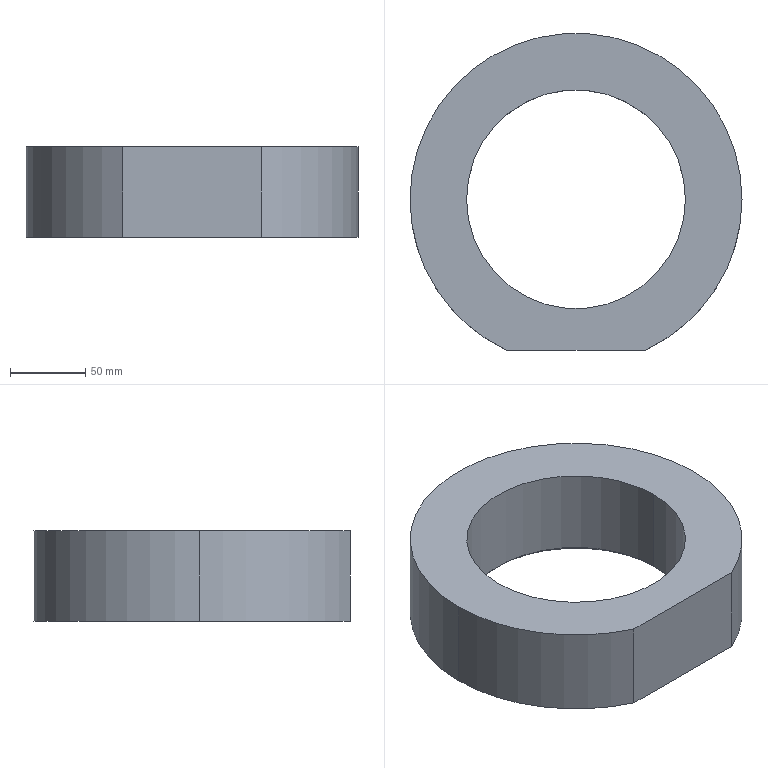Component | SolidWorks | JF21-80.1-1-3(_)-1-SOLID21-1 | 1 solid | 34 faces | box 220 x 210 x 60 mm | volume 1236758 mm3 | cylinder 17 | cone 14 | plane 3 | commonest cylinder face diameters 10.2 x12 220 x3 145 x2
STEP:
#1=CARTESIAN_POINT('',(2.854,-15.598,8.937));
#2=VERTEX_POINT('',#1);
#3=CARTESIAN_POINT('',(-2.854,-15.598,8.937));
#4=VERTEX_POINT('',#3);
#5=CARTESIAN_POINT('',(0.,-15.598,8.937));
#6=DIRECTION('',(0.,0.,-1.));
#7=DIRECTION('',(1.,0.,0.));
#8=AXIS2_PLACEMENT_3D('',#5,#6,#7);
#9=CIRCLE('',#8,2.854);
#10=EDGE_CURVE('',#2,#4,#9,.T.);
#11=ORIENTED_EDGE('',*,*,#10,.F.);
#12=CARTESIAN_POINT('',(2.933,-15.598,8.858));
#13=VERTEX_POINT('',#12);
#14=CARTESIAN_POINT('',(2.933,-15.598,8.858));
#15=DIRECTION('',(-0.7071,-0.,0.7071));
#16=VECTOR('',#15,39.37);
#17=LINE('',#14,#16);
#18=EDGE_CURVE('',#13,#2,#17,.T.);
#19=ORIENTED_EDGE('',*,*,#18,.F.);
#20=CARTESIAN_POINT('',(-2.933,-15.598,8.858));
#21=VERTEX_POINT('',#20);
#22=CARTESIAN_POINT('',(0.,-15.598,8.858));
#23=DIRECTION('',(0.,0.,1.));
#24=DIRECTION('',(1.,0.,0.));
#25=AXIS2_PLACEMENT_3D('',#22,#23,#24);
#26=CIRCLE('',#25,2.933);
#27=EDGE_CURVE('',#21,#13,#26,.T.);
#28=ORIENTED_EDGE('',*,*,#27,.F.);
#29=CARTESIAN_POINT('',(-2.933,-15.598,8.858));
#30=DIRECTION('',(0.7071,0.,0.7071));
#31=VECTOR('',#30,39.37);
#32=LINE('',#29,#31);
#33=EDGE_CURVE('',#21,#4,#32,.T.);
#34=ORIENTED_EDGE('',*,*,#33,.T.);
#35=EDGE_LOOP('',(#11,#19,#28,#34));
#36=FACE_OUTER_BOUND('',#35,.T.);
#37=CARTESIAN_POINT('',(0.,-15.598,8.858));
#38=DIRECTION('',(0.,0.,-1.));
#39=DIRECTION('',(1.,0.,0.));
#40=AXIS2_PLACEMENT_3D('',#37,#38,#39);
#41=CONICAL_SURFACE('',#40,2.933,0.7854);
#42=ADVANCED_FACE('',(#36),#41,.F.);
#43=CARTESIAN_POINT('',(3.269,-13.826,10.049));
#44=VERTEX_POINT('',#43);
#45=CARTESIAN_POINT('',(2.868,-13.826,10.049));
#46=VERTEX_POINT('',#45);
#47=CARTESIAN_POINT('',(3.069,-13.826,10.049));
#48=DIRECTION('',(0.,0.,-1.));
#49=DIRECTION('',(-1.,0.,0.));
#50=AXIS2_PLACEMENT_3D('',#47,#48,#49);
#51=CIRCLE('',#50,0.2008);
#52=EDGE_CURVE('',#44,#46,#51,.T.);
#53=ORIENTED_EDGE('',*,*,#52,.F.);
#54=CARTESIAN_POINT('',(3.269,-13.826,8.858));
#55=VERTEX_POINT('',#54);
#56=CARTESIAN_POINT('',(3.269,-13.826,8.858));
#57=DIRECTION('',(0.,0.,1.));
#58=VECTOR('',#57,39.37);
#59=LINE('',#56,#58);
#60=EDGE_CURVE('',#55,#44,#59,.T.);
#61=ORIENTED_EDGE('',*,*,#60,.F.);
#62=CARTESIAN_POINT('',(2.868,-13.826,8.858));
#63=VERTEX_POINT('',#62);
#64=CARTESIAN_POINT('',(3.069,-13.826,8.858));
#65=DIRECTION('',(0.,0.,-1.));
#66=DIRECTION('',(-1.,0.,0.));
#67=AXIS2_PLACEMENT_3D('',#64,#65,#66);
#68=CIRCLE('',#67,0.2008);
#69=EDGE_CURVE('',#55,#63,#68,.T.);
#70=ORIENTED_EDGE('',*,*,#69,.T.);
#71=CARTESIAN_POINT('',(2.868,-13.826,8.858));
#72=DIRECTION('',(0.,0.,1.));
#73=VECTOR('',#72,39.37);
#74=LINE('',#71,#73);
#75=EDGE_CURVE('',#63,#46,#74,.T.);
#76=ORIENTED_EDGE('',*,*,#75,.T.);
#77=EDGE_LOOP('',(#53,#61,#70,#76));
#78=FACE_OUTER_BOUND('',#77,.T.);
#79=CARTESIAN_POINT('',(3.069,-13.826,8.858));
#80=DIRECTION('',(0.,0.,-1.));
#81=DIRECTION('',(1.,0.,0.));
#82=AXIS2_PLACEMENT_3D('',#79,#80,#81);
#83=CYLINDRICAL_SURFACE('',#82,0.2008);
#84=ADVANCED_FACE('',(#78),#83,.F.);
#85=CARTESIAN_POINT('',(3.069,-13.826,10.17));
#86=VERTEX_POINT('',#85);
#87=CARTESIAN_POINT('',(2.868,-13.826,10.049));
#88=DIRECTION('',(0.8572,0.,0.515));
#89=VECTOR('',#88,39.37);
#90=LINE('',#87,#89);
#91=EDGE_CURVE('',#46,#86,#90,.T.);
#92=ORIENTED_EDGE('',*,*,#91,.T.);
#93=CARTESIAN_POINT('',(3.269,-13.826,10.049));
#94=DIRECTION('',(-0.8572,-0.,0.515));
#95=VECTOR('',#94,39.37);
#96=LINE('',#93,#95);
#97=EDGE_CURVE('',#44,#86,#96,.T.);
#98=ORIENTED_EDGE('',*,*,#97,.F.);
#99=ORIENTED_EDGE('',*,*,#52,.T.);
#100=EDGE_LOOP('',(#92,#98,#99));
#101=FACE_OUTER_BOUND('',#100,.T.);
#102=CARTESIAN_POINT('',(3.069,-13.826,10.049));
#103=DIRECTION('',(0.,0.,-1.));
#104=DIRECTION('',(1.,0.,0.));
#105=AXIS2_PLACEMENT_3D('',#102,#103,#104);
#106=CONICAL_SURFACE('',#105,0.2008,1.03);
#107=ADVANCED_FACE('',(#101),#106,.F.);
#108=CARTESIAN_POINT('',(3.269,-17.37,10.049));
#109=VERTEX_POINT('',#108);
#110=CARTESIAN_POINT('',(2.868,-17.37,10.049));
#111=VERTEX_POINT('',#110);
#112=CARTESIAN_POINT('',(3.069,-17.37,10.049));
#113=DIRECTION('',(0.,0.,-1.));
#114=DIRECTION('',(-1.,0.,0.));
#115=AXIS2_PLACEMENT_3D('',#112,#113,#114);
#116=CIRCLE('',#115,0.2008);
#117=EDGE_CURVE('',#109,#111,#116,.T.);
#118=ORIENTED_EDGE('',*,*,#117,.F.);
#119=CARTESIAN_POINT('',(3.269,-17.37,8.858));
#120=VERTEX_POINT('',#119);
#121=CARTESIAN_POINT('',(3.269,-17.37,8.858));
#122=DIRECTION('',(0.,0.,1.));
#123=VECTOR('',#122,39.37);
#124=LINE('',#121,#123);
#125=EDGE_CURVE('',#120,#109,#124,.T.);
#126=ORIENTED_EDGE('',*,*,#125,.F.);
#127=CARTESIAN_POINT('',(2.868,-17.37,8.858));
#128=VERTEX_POINT('',#127);
#129=CARTESIAN_POINT('',(3.069,-17.37,8.858));
#130=DIRECTION('',(0.,0.,-1.));
#131=DIRECTION('',(-1.,0.,0.));
#132=AXIS2_PLACEMENT_3D('',#129,#130,#131);
#133=CIRCLE('',#132,0.2008);
#134=EDGE_CURVE('',#120,#128,#133,.T.);
#135=ORIENTED_EDGE('',*,*,#134,.T.);
#136=CARTESIAN_POINT('',(2.868,-17.37,8.858));
#137=DIRECTION('',(0.,0.,1.));
#138=VECTOR('',#137,39.37);
#139=LINE('',#136,#138);
#140=EDGE_CURVE('',#128,#111,#139,.T.);
#141=ORIENTED_EDGE('',*,*,#140,.T.);
#142=EDGE_LOOP('',(#118,#126,#135,#141));
#143=FACE_OUTER_BOUND('',#142,.T.);
#144=CARTESIAN_POINT('',(3.069,-17.37,8.858));
#145=DIRECTION('',(0.,0.,-1.));
#146=DIRECTION('',(1.,0.,0.));
#147=AXIS2_PLACEMENT_3D('',#144,#145,#146);
#148=CYLINDRICAL_SURFACE('',#147,0.2008);
#149=ADVANCED_FACE('',(#143),#148,.F.);
#150=CARTESIAN_POINT('',(3.069,-17.37,10.17));
#151=VERTEX_POINT('',#150);
#152=CARTESIAN_POINT('',(2.868,-17.37,10.049));
#153=DIRECTION('',(0.8572,0.,0.515));
#154=VECTOR('',#153,39.37);
#155=LINE('',#152,#154);
#156=EDGE_CURVE('',#111,#151,#155,.T.);
#157=ORIENTED_EDGE('',*,*,#156,.T.);
#158=CARTESIAN_POINT('',(3.269,-17.37,10.049));
#159=DIRECTION('',(-0.8572,-0.,0.515));
#160=VECTOR('',#159,39.37);
#161=LINE('',#158,#160);
#162=EDGE_CURVE('',#109,#151,#161,.T.);
#163=ORIENTED_EDGE('',*,*,#162,.F.);
#164=ORIENTED_EDGE('',*,*,#117,.T.);
#165=EDGE_LOOP('',(#157,#163,#164));
#166=FACE_OUTER_BOUND('',#165,.T.);
#167=CARTESIAN_POINT('',(3.069,-17.37,10.049));
#168=DIRECTION('',(0.,0.,-1.));
#169=DIRECTION('',(1.,0.,0.));
#170=AXIS2_PLACEMENT_3D('',#167,#168,#169);
#171=CONICAL_SURFACE('',#170,0.2008,1.03);
#172=ADVANCED_FACE('',(#166),#171,.F.);
#173=CARTESIAN_POINT('',(0.2008,-19.141,10.049));
#174=VERTEX_POINT('',#173);
#175=CARTESIAN_POINT('',(-0.2008,-19.141,10.049));
#176=VERTEX_POINT('',#175);
#177=CARTESIAN_POINT('',(0.,-19.141,10.049));
#178=DIRECTION('',(0.,0.,-1.));
#179=DIRECTION('',(-1.,0.,0.));
#180=AXIS2_PLACEMENT_3D('',#177,#178,#179);
#181=CIRCLE('',#180,0.2008);
#182=EDGE_CURVE('',#174,#176,#181,.T.);
#183=ORIENTED_EDGE('',*,*,#182,.F.);
#184=CARTESIAN_POINT('',(0.2008,-19.141,8.858));
#185=VERTEX_POINT('',#184);
#186=CARTESIAN_POINT('',(0.2008,-19.141,8.858));
#187=DIRECTION('',(0.,0.,1.));
#188=VECTOR('',#187,39.37);
#189=LINE('',#186,#188);
#190=EDGE_CURVE('',#185,#174,#189,.T.);
#191=ORIENTED_EDGE('',*,*,#190,.F.);
#192=CARTESIAN_POINT('',(-0.2008,-19.141,8.858));
#193=VERTEX_POINT('',#192);
#194=CARTESIAN_POINT('',(0.,-19.141,8.858));
#195=DIRECTION('',(0.,0.,-1.));
#196=DIRECTION('',(-1.,0.,0.));
#197=AXIS2_PLACEMENT_3D('',#194,#195,#196);
#198=CIRCLE('',#197,0.2008);
#199=EDGE_CURVE('',#185,#193,#198,.T.);
#200=ORIENTED_EDGE('',*,*,#199,.T.);
#201=CARTESIAN_POINT('',(-0.2008,-19.141,8.858));
#202=DIRECTION('',(0.,0.,1.));
#203=VECTOR('',#202,39.37);
#204=LINE('',#201,#203);
#205=EDGE_CURVE('',#193,#176,#204,.T.);
#206=ORIENTED_EDGE('',*,*,#205,.T.);
#207=EDGE_LOOP('',(#183,#191,#200,#206));
#208=FACE_OUTER_BOUND('',#207,.T.);
#209=CARTESIAN_POINT('',(0.,-19.141,8.858));
#210=DIRECTION('',(0.,0.,-1.));
#211=DIRECTION('',(1.,0.,0.));
#212=AXIS2_PLACEMENT_3D('',#209,#210,#211);
#213=CYLINDRICAL_SURFACE('',#212,0.2008);
#214=ADVANCED_FACE('',(#208),#213,.F.);
#215=CARTESIAN_POINT('',(0.,-19.141,10.17));
#216=VERTEX_POINT('',#215);
#217=CARTESIAN_POINT('',(-0.2008,-19.141,10.049));
#218=DIRECTION('',(0.8572,0.,0.515));
#219=VECTOR('',#218,39.37);
#220=LINE('',#217,#219);
#221=EDGE_CURVE('',#176,#216,#220,.T.);
#222=ORIENTED_EDGE('',*,*,#221,.T.);
#223=CARTESIAN_POINT('',(0.2008,-19.141,10.049));
#224=DIRECTION('',(-0.8572,-0.,0.515));
#225=VECTOR('',#224,39.37);
#226=LINE('',#223,#225);
#227=EDGE_CURVE('',#174,#216,#226,.T.);
#228=ORIENTED_EDGE('',*,*,#227,.F.);
#229=ORIENTED_EDGE('',*,*,#182,.T.);
#230=EDGE_LOOP('',(#222,#228,#229));
#231=FACE_OUTER_BOUND('',#230,.T.);
#232=CARTESIAN_POINT('',(0.,-19.141,10.049));
#233=DIRECTION('',(0.,0.,-1.));
#234=DIRECTION('',(1.,0.,0.));
#235=AXIS2_PLACEMENT_3D('',#232,#233,#234);
#236=CONICAL_SURFACE('',#235,0.2008,1.03);
#237=ADVANCED_FACE('',(#231),#236,.F.);
#238=CARTESIAN_POINT('',(-2.868,-17.37,10.049));
#239=VERTEX_POINT('',#238);
#240=CARTESIAN_POINT('',(-3.269,-17.37,10.049));
#241=VERTEX_POINT('',#240);
#242=CARTESIAN_POINT('',(-3.069,-17.37,10.049));
#243=DIRECTION('',(0.,0.,-1.));
#244=DIRECTION('',(-1.,0.,0.));
#245=AXIS2_PLACEMENT_3D('',#242,#243,#244);
#246=CIRCLE('',#245,0.2008);
#247=EDGE_CURVE('',#239,#241,#246,.T.);
#248=ORIENTED_EDGE('',*,*,#247,.F.);
#249=CARTESIAN_POINT('',(-2.868,-17.37,8.858));
#250=VERTEX_POINT('',#249);
#251=CARTESIAN_POINT('',(-2.868,-17.37,8.858));
#252=DIRECTION('',(0.,0.,1.));
#253=VECTOR('',#252,39.37);
#254=LINE('',#251,#253);
#255=EDGE_CURVE('',#250,#239,#254,.T.);
#256=ORIENTED_EDGE('',*,*,#255,.F.);
#257=CARTESIAN_POINT('',(-3.269,-17.37,8.858));
#258=VERTEX_POINT('',#257);
#259=CARTESIAN_POINT('',(-3.069,-17.37,8.858));
#260=DIRECTION('',(0.,0.,-1.));
#261=DIRECTION('',(-1.,0.,0.));
#262=AXIS2_PLACEMENT_3D('',#259,#260,#261);
#263=CIRCLE('',#262,0.2008);
#264=EDGE_CURVE('',#250,#258,#263,.T.);
#265=ORIENTED_EDGE('',*,*,#264,.T.);
#266=CARTESIAN_POINT('',(-3.269,-17.37,8.858));
#267=DIRECTION('',(0.,0.,1.));
#268=VECTOR('',#267,39.37);
#269=LINE('',#266,#268);
#270=EDGE_CURVE('',#258,#241,#269,.T.);
#271=ORIENTED_EDGE('',*,*,#270,.T.);
#272=EDGE_LOOP('',(#248,#256,#265,#271));
#273=FACE_OUTER_BOUND('',#272,.T.);
#274=CARTESIAN_POINT('',(-3.069,-17.37,8.858));
#275=DIRECTION('',(0.,0.,-1.));
#276=DIRECTION('',(1.,0.,0.));
#277=AXIS2_PLACEMENT_3D('',#274,#275,#276);
#278=CYLINDRICAL_SURFACE('',#277,0.2008);
#279=ADVANCED_FACE('',(#273),#278,.F.);
#280=CARTESIAN_POINT('',(-3.069,-17.37,10.17));
#281=VERTEX_POINT('',#280);
#282=CARTESIAN_POINT('',(-3.269,-17.37,10.049));
#283=DIRECTION('',(0.8572,0.,0.515));
#284=VECTOR('',#283,39.37);
#285=LINE('',#282,#284);
#286=EDGE_CURVE('',#241,#281,#285,.T.);
#287=ORIENTED_EDGE('',*,*,#286,.T.);
#288=CARTESIAN_POINT('',(-2.868,-17.37,10.049));
#289=DIRECTION('',(-0.8572,-0.,0.515));
#290=VECTOR('',#289,39.37);
#291=LINE('',#288,#290);
#292=EDGE_CURVE('',#239,#281,#291,.T.);
#293=ORIENTED_EDGE('',*,*,#292,.F.);
#294=ORIENTED_EDGE('',*,*,#247,.T.);
#295=EDGE_LOOP('',(#287,#293,#294));
#296=FACE_OUTER_BOUND('',#295,.T.);
#297=CARTESIAN_POINT('',(-3.069,-17.37,10.049));
#298=DIRECTION('',(0.,0.,-1.));
#299=DIRECTION('',(1.,0.,0.));
#300=AXIS2_PLACEMENT_3D('',#297,#298,#299);
#301=CONICAL_SURFACE('',#300,0.2008,1.03);
#302=ADVANCED_FACE('',(#296),#301,.F.);
#303=CARTESIAN_POINT('',(-2.868,-13.826,10.049));
#304=VERTEX_POINT('',#303);
#305=CARTESIAN_POINT('',(-3.269,-13.826,10.049));
#306=VERTEX_POINT('',#305);
#307=CARTESIAN_POINT('',(-3.069,-13.826,10.049));
#308=DIRECTION('',(0.,0.,-1.));
#309=DIRECTION('',(-1.,0.,0.));
#310=AXIS2_PLACEMENT_3D('',#307,#308,#309);
#311=CIRCLE('',#310,0.2008);
#312=EDGE_CURVE('',#304,#306,#311,.T.);
#313=ORIENTED_EDGE('',*,*,#312,.F.);
#314=CARTESIAN_POINT('',(-2.868,-13.826,8.858));
#315=VERTEX_POINT('',#314);
#316=CARTESIAN_POINT('',(-2.868,-13.826,8.858));
#317=DIRECTION('',(0.,0.,1.));
#318=VECTOR('',#317,39.37);
#319=LINE('',#316,#318);
#320=EDGE_CURVE('',#315,#304,#319,.T.);
#321=ORIENTED_EDGE('',*,*,#320,.F.);
#322=CARTESIAN_POINT('',(-3.269,-13.826,8.858));
#323=VERTEX_POINT('',#322);
#324=CARTESIAN_POINT('',(-3.069,-13.826,8.858));
#325=DIRECTION('',(0.,0.,-1.));
#326=DIRECTION('',(-1.,0.,0.));
#327=AXIS2_PLACEMENT_3D('',#324,#325,#326);
#328=CIRCLE('',#327,0.2008);
#329=EDGE_CURVE('',#315,#323,#328,.T.);
#330=ORIENTED_EDGE('',*,*,#329,.T.);
#331=CARTESIAN_POINT('',(-3.269,-13.826,8.858));
#332=DIRECTION('',(0.,0.,1.));
#333=VECTOR('',#332,39.37);
#334=LINE('',#331,#333);
#335=EDGE_CURVE('',#323,#306,#334,.T.);
#336=ORIENTED_EDGE('',*,*,#335,.T.);
#337=EDGE_LOOP('',(#313,#321,#330,#336));
#338=FACE_OUTER_BOUND('',#337,.T.);
#339=CARTESIAN_POINT('',(-3.069,-13.826,8.858));
#340=DIRECTION('',(0.,0.,-1.));
#341=DIRECTION('',(1.,0.,0.));
#342=AXIS2_PLACEMENT_3D('',#339,#340,#341);
#343=CYLINDRICAL_SURFACE('',#342,0.2008);
#344=ADVANCED_FACE('',(#338),#343,.F.);
#345=CARTESIAN_POINT('',(-3.069,-13.826,10.17));
#346=VERTEX_POINT('',#345);
#347=CARTESIAN_POINT('',(-3.269,-13.826,10.049));
#348=DIRECTION('',(0.8572,0.,0.515));
#349=VECTOR('',#348,39.37);
#350=LINE('',#347,#349);
#351=EDGE_CURVE('',#306,#346,#350,.T.);
#352=ORIENTED_EDGE('',*,*,#351,.T.);
#353=CARTESIAN_POINT('',(-2.868,-13.826,10.049));
#354=DIRECTION('',(-0.8572,-0.,0.515));
#355=VECTOR('',#354,39.37);
#356=LINE('',#353,#355);
#357=EDGE_CURVE('',#304,#346,#356,.T.);
#358=ORIENTED_EDGE('',*,*,#357,.F.);
#359=ORIENTED_EDGE('',*,*,#312,.T.);
#360=EDGE_LOOP('',(#352,#358,#359));
#361=FACE_OUTER_BOUND('',#360,.T.);
#362=CARTESIAN_POINT('',(-3.069,-13.826,10.049));
#363=DIRECTION('',(0.,0.,-1.));
#364=DIRECTION('',(1.,0.,0.));
#365=AXIS2_PLACEMENT_3D('',#362,#363,#364);
#366=CONICAL_SURFACE('',#365,0.2008,1.03);
#367=ADVANCED_FACE('',(#361),#366,.F.);
#368=CARTESIAN_POINT('',(0.2008,-12.055,10.049));
#369=VERTEX_POINT('',#368);
#370=CARTESIAN_POINT('',(-0.2008,-12.055,10.049));
#371=VERTEX_POINT('',#370);
#372=CARTESIAN_POINT('',(0.,-12.055,10.049));
#373=DIRECTION('',(0.,0.,-1.));
#374=DIRECTION('',(-1.,0.,0.));
#375=AXIS2_PLACEMENT_3D('',#372,#373,#374);
#376=CIRCLE('',#375,0.2008);
#377=EDGE_CURVE('',#369,#371,#376,.T.);
#378=ORIENTED_EDGE('',*,*,#377,.F.);
#379=CARTESIAN_POINT('',(0.2008,-12.055,8.858));
#380=VERTEX_POINT('',#379);
#381=CARTESIAN_POINT('',(0.2008,-12.055,8.858));
#382=DIRECTION('',(0.,0.,1.));
#383=VECTOR('',#382,39.37);
#384=LINE('',#381,#383);
#385=EDGE_CURVE('',#380,#369,#384,.T.);
#386=ORIENTED_EDGE('',*,*,#385,.F.);
#387=CARTESIAN_POINT('',(-0.2008,-12.055,8.858));
#388=VERTEX_POINT('',#387);
#389=CARTESIAN_POINT('',(0.,-12.055,8.858));
#390=DIRECTION('',(0.,0.,-1.));
#391=DIRECTION('',(-1.,0.,0.));
#392=AXIS2_PLACEMENT_3D('',#389,#390,#391);
#393=CIRCLE('',#392,0.2008);
#394=EDGE_CURVE('',#380,#388,#393,.T.);
#395=ORIENTED_EDGE('',*,*,#394,.T.);
#396=CARTESIAN_POINT('',(-0.2008,-12.055,8.858));
#397=DIRECTION('',(0.,0.,1.));
#398=VECTOR('',#397,39.37);
#399=LINE('',#396,#398);
#400=EDGE_CURVE('',#388,#371,#399,.T.);
#401=ORIENTED_EDGE('',*,*,#400,.T.);
#402=EDGE_LOOP('',(#378,#386,#395,#401));
#403=FACE_OUTER_BOUND('',#402,.T.);
#404=CARTESIAN_POINT('',(0.,-12.055,8.858));
#405=DIRECTION('',(0.,0.,-1.));
#406=DIRECTION('',(1.,0.,0.));
#407=AXIS2_PLACEMENT_3D('',#404,#405,#406);
#408=CYLINDRICAL_SURFACE('',#407,0.2008);
#409=ADVANCED_FACE('',(#403),#408,.F.);
#410=CARTESIAN_POINT('',(-0.,-12.055,10.17));
#411=VERTEX_POINT('',#410);
#412=CARTESIAN_POINT('',(-0.2008,-12.055,10.049));
#413=DIRECTION('',(0.8572,0.,0.515));
#414=VECTOR('',#413,39.37);
#415=LINE('',#412,#414);
#416=EDGE_CURVE('',#371,#411,#415,.T.);
#417=ORIENTED_EDGE('',*,*,#416,.T.);
#418=CARTESIAN_POINT('',(0.2008,-12.055,10.049));
#419=DIRECTION('',(-0.8572,-0.,0.515));
#420=VECTOR('',#419,39.37);
#421=LINE('',#418,#420);
#422=EDGE_CURVE('',#369,#411,#421,.T.);
#423=ORIENTED_EDGE('',*,*,#422,.F.);
#424=ORIENTED_EDGE('',*,*,#377,.T.);
#425=EDGE_LOOP('',(#417,#423,#424));
#426=FACE_OUTER_BOUND('',#425,.T.);
#427=CARTESIAN_POINT('',(0.,-12.055,10.049));
#428=DIRECTION('',(0.,0.,-1.));
#429=DIRECTION('',(1.,0.,0.));
#430=AXIS2_PLACEMENT_3D('',#427,#428,#429);
#431=CONICAL_SURFACE('',#430,0.2008,1.03);
#432=ADVANCED_FACE('',(#426),#431,.F.);
#433=ORIENTED_EDGE('',*,*,#10,.T.);
#434=CARTESIAN_POINT('',(-2.854,-15.598,11.22));
#435=VERTEX_POINT('',#434);
#436=CARTESIAN_POINT('',(-2.854,-15.598,8.858));
#437=DIRECTION('',(0.,0.,1.));
#438=VECTOR('',#437,39.37);
#439=LINE('',#436,#438);
#440=EDGE_CURVE('',#4,#435,#439,.T.);
#441=ORIENTED_EDGE('',*,*,#440,.T.);
#442=CARTESIAN_POINT('',(2.854,-15.598,11.22));
#443=VERTEX_POINT('',#442);
#444=CARTESIAN_POINT('',(0.,-15.598,11.22));
#445=DIRECTION('',(0.,0.,1.));
#446=DIRECTION('',(1.,0.,0.));
#447=AXIS2_PLACEMENT_3D('',#444,#445,#446);
#448=CIRCLE('',#447,2.854);
#449=EDGE_CURVE('',#435,#443,#448,.T.);
#450=ORIENTED_EDGE('',*,*,#449,.T.);
#451=CARTESIAN_POINT('',(2.854,-15.598,8.858));
#452=DIRECTION('',(0.,0.,1.));
#453=VECTOR('',#452,39.37);
#454=LINE('',#451,#453);
#455=EDGE_CURVE('',#2,#443,#454,.T.);
#456=ORIENTED_EDGE('',*,*,#455,.F.);
#457=EDGE_LOOP('',(#433,#441,#450,#456));
#458=FACE_OUTER_BOUND('',#457,.T.);
#459=CARTESIAN_POINT('',(0.,-15.598,8.858));
#460=DIRECTION('',(0.,0.,1.));
#461=DIRECTION('',(-1.,0.,0.));
#462=AXIS2_PLACEMENT_3D('',#459,#460,#461);
#463=CYLINDRICAL_SURFACE('',#462,2.854);
#464=ADVANCED_FACE('',(#458),#463,.F.);
#465=CARTESIAN_POINT('',(4.331,-15.598,8.858));
#466=VERTEX_POINT('',#465);
#467=CARTESIAN_POINT('',(-4.331,-15.598,8.858));
#468=VERTEX_POINT('',#467);
#469=CARTESIAN_POINT('',(0.,-15.598,8.858));
#470=DIRECTION('',(0.,0.,1.));
#471=DIRECTION('',(1.,0.,0.));
#472=AXIS2_PLACEMENT_3D('',#469,#470,#471);
#473=CIRCLE('',#472,4.331);
#474=EDGE_CURVE('',#466,#468,#473,.T.);
#475=ORIENTED_EDGE('',*,*,#474,.T.);
#476=CARTESIAN_POINT('',(-4.331,-15.598,11.22));
#477=VERTEX_POINT('',#476);
#478=CARTESIAN_POINT('',(-4.331,-15.598,8.858));
#479=DIRECTION('',(0.,0.,1.));
#480=VECTOR('',#479,39.37);
#481=LINE('',#478,#480);
#482=EDGE_CURVE('',#468,#477,#481,.T.);
#483=ORIENTED_EDGE('',*,*,#482,.T.);
#484=CARTESIAN_POINT('',(4.331,-15.598,11.22));
#485=VERTEX_POINT('',#484);
#486=CARTESIAN_POINT('',(0.,-15.598,11.22));
#487=DIRECTION('',(0.,0.,1.));
#488=DIRECTION('',(1.,0.,0.));
#489=AXIS2_PLACEMENT_3D('',#486,#487,#488);
#490=CIRCLE('',#489,4.331);
#491=EDGE_CURVE('',#485,#477,#490,.T.);
#492=ORIENTED_EDGE('',*,*,#491,.F.);
#493=CARTESIAN_POINT('',(4.331,-15.598,8.858));
#494=DIRECTION('',(0.,0.,1.));
#495=VECTOR('',#494,39.37);
#496=LINE('',#493,#495);
#497=EDGE_CURVE('',#466,#485,#496,.T.);
#498=ORIENTED_EDGE('',*,*,#497,.F.);
#499=EDGE_LOOP('',(#475,#483,#492,#498));
#500=FACE_OUTER_BOUND('',#499,.T.);
#501=CARTESIAN_POINT('',(0.,-15.598,8.858));
#502=DIRECTION('',(0.,0.,1.));
#503=DIRECTION('',(-1.,0.,0.));
#504=AXIS2_PLACEMENT_3D('',#501,#502,#503);
#505=CYLINDRICAL_SURFACE('',#504,4.331);
#506=ADVANCED_FACE('',(#500),#505,.T.);
#507=CARTESIAN_POINT('',(1.804,-19.535,8.858));
#508=VERTEX_POINT('',#507);
#509=CARTESIAN_POINT('',(0.,-15.598,8.858));
#510=DIRECTION('',(0.,0.,1.));
#511=DIRECTION('',(1.,0.,0.));
#512=AXIS2_PLACEMENT_3D('',#509,#510,#511);
#513=CIRCLE('',#512,4.331);
#514=EDGE_CURVE('',#508,#466,#513,.T.);
#515=ORIENTED_EDGE('',*,*,#514,.T.);
#516=ORIENTED_EDGE('',*,*,#497,.T.);
#517=CARTESIAN_POINT('',(1.804,-19.535,11.22));
#518=VERTEX_POINT('',#517);
#519=CARTESIAN_POINT('',(0.,-15.598,11.22));
#520=DIRECTION('',(0.,0.,1.));
#521=DIRECTION('',(1.,0.,0.));
#522=AXIS2_PLACEMENT_3D('',#519,#520,#521);
#523=CIRCLE('',#522,4.331);
#524=EDGE_CURVE('',#518,#485,#523,.T.);
#525=ORIENTED_EDGE('',*,*,#524,.F.);
#526=CARTESIAN_POINT('',(1.804,-19.535,8.858));
#527=DIRECTION('',(0.,0.,1.));
#528=VECTOR('',#527,39.37);
#529=LINE('',#526,#528);
#530=EDGE_CURVE('',#508,#518,#529,.T.);
#531=ORIENTED_EDGE('',*,*,#530,.F.);
#532=EDGE_LOOP('',(#515,#516,#525,#531));
#533=FACE_OUTER_BOUND('',#532,.T.);
#534=CARTESIAN_POINT('',(0.,-15.598,8.858));
#535=DIRECTION('',(0.,0.,1.));
#536=DIRECTION('',(-1.,0.,0.));
#537=AXIS2_PLACEMENT_3D('',#534,#535,#536);
#538=CYLINDRICAL_SURFACE('',#537,4.331);
#539=ADVANCED_FACE('',(#533),#538,.T.);
#540=ORIENTED_EDGE('',*,*,#482,.F.);
#541=CARTESIAN_POINT('',(-1.804,-19.535,8.858));
#542=VERTEX_POINT('',#541);
#543=CARTESIAN_POINT('',(0.,-15.598,8.858));
#544=DIRECTION('',(0.,0.,1.));
#545=DIRECTION('',(1.,0.,0.));
#546=AXIS2_PLACEMENT_3D('',#543,#544,#545);
#547=CIRCLE('',#546,4.331);
#548=EDGE_CURVE('',#468,#542,#547,.T.);
#549=ORIENTED_EDGE('',*,*,#548,.T.);
#550=CARTESIAN_POINT('',(-1.804,-19.535,11.22));
#551=VERTEX_POINT('',#550);
#552=CARTESIAN_POINT('',(-1.804,-19.535,8.858));
#553=DIRECTION('',(0.,0.,1.));
#554=VECTOR('',#553,39.37);
#555=LINE('',#552,#554);
#556=EDGE_CURVE('',#542,#551,#555,.T.);
#557=ORIENTED_EDGE('',*,*,#556,.T.);
#558=CARTESIAN_POINT('',(0.,-15.598,11.22));
#559=DIRECTION('',(0.,0.,1.));
#560=DIRECTION('',(1.,0.,0.));
#561=AXIS2_PLACEMENT_3D('',#558,#559,#560);
#562=CIRCLE('',#561,4.331);
#563=EDGE_CURVE('',#477,#551,#562,.T.);
#564=ORIENTED_EDGE('',*,*,#563,.F.);
#565=EDGE_LOOP('',(#540,#549,#557,#564));
#566=FACE_OUTER_BOUND('',#565,.T.);
#567=CARTESIAN_POINT('',(0.,-15.598,8.858));
#568=DIRECTION('',(0.,0.,1.));
#569=DIRECTION('',(-1.,0.,0.));
#570=AXIS2_PLACEMENT_3D('',#567,#568,#569);
#571=CYLINDRICAL_SURFACE('',#570,4.331);
#572=ADVANCED_FACE('',(#566),#571,.T.);
#573=CARTESIAN_POINT('',(-1.804,-19.535,11.22));
#574=DIRECTION('',(1.,-0.,0.));
#575=VECTOR('',#574,39.37);
#576=LINE('',#573,#575);
#577=EDGE_CURVE('',#551,#518,#576,.T.);
#578=ORIENTED_EDGE('',*,*,#577,.F.);
#579=ORIENTED_EDGE('',*,*,#556,.F.);
#580=CARTESIAN_POINT('',(-1.804,-19.535,8.858));
#581=DIRECTION('',(1.,-0.,0.));
#582=VECTOR('',#581,39.37);
#583=LINE('',#580,#582);
#584=EDGE_CURVE('',#542,#508,#583,.T.);
#585=ORIENTED_EDGE('',*,*,#584,.T.);
#586=ORIENTED_EDGE('',*,*,#530,.T.);
#587=EDGE_LOOP('',(#578,#579,#585,#586));
#588=FACE_OUTER_BOUND('',#587,.T.);
#589=CARTESIAN_POINT('',(-1.804,-19.535,8.858));
#590=DIRECTION('',(-0.,-1.,0.));
#591=DIRECTION('',(-1.,0.,0.));
#592=AXIS2_PLACEMENT_3D('',#589,#590,#591);
#593=PLANE('',#592);
#594=ADVANCED_FACE('',(#588),#593,.T.);
#595=ORIENTED_EDGE('',*,*,#27,.T.);
#596=CARTESIAN_POINT('',(0.,-15.598,8.858));
#597=DIRECTION('',(0.,0.,1.));
#598=DIRECTION('',(1.,0.,0.));
#599=AXIS2_PLACEMENT_3D('',#596,#597,#598);
#600=CIRCLE('',#599,2.933);
#601=EDGE_CURVE('',#13,#21,#600,.T.);
#602=ORIENTED_EDGE('',*,*,#601,.T.);
#603=EDGE_LOOP('',(#595,#602));
#604=FACE_BOUND('',#603,.T.);
#605=CARTESIAN_POINT('',(3.069,-13.826,8.858));
#606=DIRECTION('',(0.,0.,-1.));
#607=DIRECTION('',(-1.,0.,0.));
#608=AXIS2_PLACEMENT_3D('',#605,#606,#607);
#609=CIRCLE('',#608,0.2008);
#610=EDGE_CURVE('',#63,#55,#609,.T.);
#611=ORIENTED_EDGE('',*,*,#610,.F.);
#612=ORIENTED_EDGE('',*,*,#69,.F.);
#613=EDGE_LOOP('',(#611,#612));
#614=FACE_BOUND('',#613,.T.);
#615=CARTESIAN_POINT('',(3.069,-17.37,8.858));
#616=DIRECTION('',(0.,0.,-1.));
#617=DIRECTION('',(-1.,0.,0.));
#618=AXIS2_PLACEMENT_3D('',#615,#616,#617);
#619=CIRCLE('',#618,0.2008);
#620=EDGE_CURVE('',#128,#120,#619,.T.);
#621=ORIENTED_EDGE('',*,*,#620,.F.);
#622=ORIENTED_EDGE('',*,*,#134,.F.);
#623=EDGE_LOOP('',(#621,#622));
#624=FACE_BOUND('',#623,.T.);
#625=CARTESIAN_POINT('',(0.,-19.141,8.858));
#626=DIRECTION('',(0.,0.,-1.));
#627=DIRECTION('',(-1.,0.,0.));
#628=AXIS2_PLACEMENT_3D('',#625,#626,#627);
#629=CIRCLE('',#628,0.2008);
#630=EDGE_CURVE('',#193,#185,#629,.T.);
#631=ORIENTED_EDGE('',*,*,#630,.F.);
#632=ORIENTED_EDGE('',*,*,#199,.F.);
#633=EDGE_LOOP('',(#631,#632));
#634=FACE_BOUND('',#633,.T.);
#635=CARTESIAN_POINT('',(-3.069,-17.37,8.858));
#636=DIRECTION('',(0.,0.,-1.));
#637=DIRECTION('',(-1.,0.,0.));
#638=AXIS2_PLACEMENT_3D('',#635,#636,#637);
#639=CIRCLE('',#638,0.2008);
#640=EDGE_CURVE('',#258,#250,#639,.T.);
#641=ORIENTED_EDGE('',*,*,#640,.F.);
#642=ORIENTED_EDGE('',*,*,#264,.F.);
#643=EDGE_LOOP('',(#641,#642));
#644=FACE_BOUND('',#643,.T.);
#645=CARTESIAN_POINT('',(-3.069,-13.826,8.858));
#646=DIRECTION('',(0.,0.,-1.));
#647=DIRECTION('',(-1.,0.,0.));
#648=AXIS2_PLACEMENT_3D('',#645,#646,#647);
#649=CIRCLE('',#648,0.2008);
#650=EDGE_CURVE('',#323,#315,#649,.T.);
#651=ORIENTED_EDGE('',*,*,#650,.F.);
#652=ORIENTED_EDGE('',*,*,#329,.F.);
#653=EDGE_LOOP('',(#651,#652));
#654=FACE_BOUND('',#653,.T.);
#655=CARTESIAN_POINT('',(0.,-12.055,8.858));
#656=DIRECTION('',(0.,0.,-1.));
#657=DIRECTION('',(-1.,0.,0.));
#658=AXIS2_PLACEMENT_3D('',#655,#656,#657);
#659=CIRCLE('',#658,0.2008);
#660=EDGE_CURVE('',#388,#380,#659,.T.);
#661=ORIENTED_EDGE('',*,*,#660,.F.);
#662=ORIENTED_EDGE('',*,*,#394,.F.);
#663=EDGE_LOOP('',(#661,#662));
#664=FACE_BOUND('',#663,.T.);
#665=ORIENTED_EDGE('',*,*,#514,.F.);
#666=ORIENTED_EDGE('',*,*,#584,.F.);
#667=ORIENTED_EDGE('',*,*,#548,.F.);
#668=ORIENTED_EDGE('',*,*,#474,.F.);
#669=EDGE_LOOP('',(#665,#666,#667,#668));
#670=FACE_OUTER_BOUND('',#669,.T.);
#671=CARTESIAN_POINT('',(0.,-15.598,8.858));
#672=DIRECTION('',(0.,0.,1.));
#673=DIRECTION('',(-1.,0.,0.));
#674=AXIS2_PLACEMENT_3D('',#671,#672,#673);
#675=PLANE('',#674);
#676=ADVANCED_FACE('',(#604,#614,#624,#634,#644,#654,#664,#670),#675,.F.);
#677=CARTESIAN_POINT('',(0.,-15.598,11.22));
#678=DIRECTION('',(0.,0.,1.));
#679=DIRECTION('',(1.,0.,0.));
#680=AXIS2_PLACEMENT_3D('',#677,#678,#679);
#681=CIRCLE('',#680,2.854);
#682=EDGE_CURVE('',#443,#435,#681,.T.);
#683=ORIENTED_EDGE('',*,*,#682,.F.);
#684=ORIENTED_EDGE('',*,*,#449,.F.);
#685=EDGE_LOOP('',(#683,#684));
#686=FACE_BOUND('',#685,.T.);
#687=ORIENTED_EDGE('',*,*,#524,.T.);
#688=ORIENTED_EDGE('',*,*,#491,.T.);
#689=ORIENTED_EDGE('',*,*,#563,.T.);
#690=ORIENTED_EDGE('',*,*,#577,.T.);
#691=EDGE_LOOP('',(#687,#688,#689,#690));
#692=FACE_OUTER_BOUND('',#691,.T.);
#693=CARTESIAN_POINT('',(0.,-15.598,11.22));
#694=DIRECTION('',(0.,0.,1.));
#695=DIRECTION('',(-1.,0.,0.));
#696=AXIS2_PLACEMENT_3D('',#693,#694,#695);
#697=PLANE('',#696);
#698=ADVANCED_FACE('',(#686,#692),#697,.T.);
#699=ORIENTED_EDGE('',*,*,#440,.F.);
#700=CARTESIAN_POINT('',(0.,-15.598,8.937));
#701=DIRECTION('',(0.,0.,-1.));
#702=DIRECTION('',(1.,0.,0.));
#703=AXIS2_PLACEMENT_3D('',#700,#701,#702);
#704=CIRCLE('',#703,2.854);
#705=EDGE_CURVE('',#4,#2,#704,.T.);
#706=ORIENTED_EDGE('',*,*,#705,.T.);
#707=ORIENTED_EDGE('',*,*,#455,.T.);
#708=ORIENTED_EDGE('',*,*,#682,.T.);
#709=EDGE_LOOP('',(#699,#706,#707,#708));
#710=FACE_OUTER_BOUND('',#709,.T.);
#711=CARTESIAN_POINT('',(0.,-15.598,8.858));
#712=DIRECTION('',(0.,0.,1.));
#713=DIRECTION('',(-1.,0.,0.));
#714=AXIS2_PLACEMENT_3D('',#711,#712,#713);
#715=CYLINDRICAL_SURFACE('',#714,2.854);
#716=ADVANCED_FACE('',(#710),#715,.F.);
#717=ORIENTED_EDGE('',*,*,#422,.T.);
#718=ORIENTED_EDGE('',*,*,#416,.F.);
#719=CARTESIAN_POINT('',(0.,-12.055,10.049));
#720=DIRECTION('',(0.,0.,-1.));
#721=DIRECTION('',(-1.,0.,0.));
#722=AXIS2_PLACEMENT_3D('',#719,#720,#721);
#723=CIRCLE('',#722,0.2008);
#724=EDGE_CURVE('',#371,#369,#723,.T.);
#725=ORIENTED_EDGE('',*,*,#724,.T.);
#726=EDGE_LOOP('',(#717,#718,#725));
#727=FACE_OUTER_BOUND('',#726,.T.);
#728=CARTESIAN_POINT('',(0.,-12.055,10.049));
#729=DIRECTION('',(0.,0.,-1.));
#730=DIRECTION('',(1.,0.,0.));
#731=AXIS2_PLACEMENT_3D('',#728,#729,#730);
#732=CONICAL_SURFACE('',#731,0.2008,1.03);
#733=ADVANCED_FACE('',(#727),#732,.F.);
#734=ORIENTED_EDGE('',*,*,#385,.T.);
#735=ORIENTED_EDGE('',*,*,#724,.F.);
#736=ORIENTED_EDGE('',*,*,#400,.F.);
#737=ORIENTED_EDGE('',*,*,#660,.T.);
#738=EDGE_LOOP('',(#734,#735,#736,#737));
#739=FACE_OUTER_BOUND('',#738,.T.);
#740=CARTESIAN_POINT('',(0.,-12.055,8.858));
#741=DIRECTION('',(0.,0.,-1.));
#742=DIRECTION('',(1.,0.,0.));
#743=AXIS2_PLACEMENT_3D('',#740,#741,#742);
#744=CYLINDRICAL_SURFACE('',#743,0.2008);
#745=ADVANCED_FACE('',(#739),#744,.F.);
#746=ORIENTED_EDGE('',*,*,#357,.T.);
#747=ORIENTED_EDGE('',*,*,#351,.F.);
#748=CARTESIAN_POINT('',(-3.069,-13.826,10.049));
#749=DIRECTION('',(0.,0.,-1.));
#750=DIRECTION('',(-1.,0.,0.));
#751=AXIS2_PLACEMENT_3D('',#748,#749,#750);
#752=CIRCLE('',#751,0.2008);
#753=EDGE_CURVE('',#306,#304,#752,.T.);
#754=ORIENTED_EDGE('',*,*,#753,.T.);
#755=EDGE_LOOP('',(#746,#747,#754));
#756=FACE_OUTER_BOUND('',#755,.T.);
#757=CARTESIAN_POINT('',(-3.069,-13.826,10.049));
#758=DIRECTION('',(0.,0.,-1.));
#759=DIRECTION('',(1.,0.,0.));
#760=AXIS2_PLACEMENT_3D('',#757,#758,#759);
#761=CONICAL_SURFACE('',#760,0.2008,1.03);
#762=ADVANCED_FACE('',(#756),#761,.F.);
#763=ORIENTED_EDGE('',*,*,#320,.T.);
#764=ORIENTED_EDGE('',*,*,#753,.F.);
#765=ORIENTED_EDGE('',*,*,#335,.F.);
#766=ORIENTED_EDGE('',*,*,#650,.T.);
#767=EDGE_LOOP('',(#763,#764,#765,#766));
#768=FACE_OUTER_BOUND('',#767,.T.);
#769=CARTESIAN_POINT('',(-3.069,-13.826,8.858));
#770=DIRECTION('',(0.,0.,-1.));
#771=DIRECTION('',(1.,0.,0.));
#772=AXIS2_PLACEMENT_3D('',#769,#770,#771);
#773=CYLINDRICAL_SURFACE('',#772,0.2008);
#774=ADVANCED_FACE('',(#768),#773,.F.);
#775=ORIENTED_EDGE('',*,*,#292,.T.);
#776=ORIENTED_EDGE('',*,*,#286,.F.);
#777=CARTESIAN_POINT('',(-3.069,-17.37,10.049));
#778=DIRECTION('',(0.,0.,-1.));
#779=DIRECTION('',(-1.,0.,0.));
#780=AXIS2_PLACEMENT_3D('',#777,#778,#779);
#781=CIRCLE('',#780,0.2008);
#782=EDGE_CURVE('',#241,#239,#781,.T.);
#783=ORIENTED_EDGE('',*,*,#782,.T.);
#784=EDGE_LOOP('',(#775,#776,#783));
#785=FACE_OUTER_BOUND('',#784,.T.);
#786=CARTESIAN_POINT('',(-3.069,-17.37,10.049));
#787=DIRECTION('',(0.,0.,-1.));
#788=DIRECTION('',(1.,0.,0.));
#789=AXIS2_PLACEMENT_3D('',#786,#787,#788);
#790=CONICAL_SURFACE('',#789,0.2008,1.03);
#791=ADVANCED_FACE('',(#785),#790,.F.);
#792=ORIENTED_EDGE('',*,*,#255,.T.);
#793=ORIENTED_EDGE('',*,*,#782,.F.);
#794=ORIENTED_EDGE('',*,*,#270,.F.);
#795=ORIENTED_EDGE('',*,*,#640,.T.);
#796=EDGE_LOOP('',(#792,#793,#794,#795));
#797=FACE_OUTER_BOUND('',#796,.T.);
#798=CARTESIAN_POINT('',(-3.069,-17.37,8.858));
#799=DIRECTION('',(0.,0.,-1.));
#800=DIRECTION('',(1.,0.,0.));
#801=AXIS2_PLACEMENT_3D('',#798,#799,#800);
#802=CYLINDRICAL_SURFACE('',#801,0.2008);
#803=ADVANCED_FACE('',(#797),#802,.F.);
#804=ORIENTED_EDGE('',*,*,#227,.T.);
#805=ORIENTED_EDGE('',*,*,#221,.F.);
#806=CARTESIAN_POINT('',(0.,-19.141,10.049));
#807=DIRECTION('',(0.,0.,-1.));
#808=DIRECTION('',(-1.,0.,0.));
#809=AXIS2_PLACEMENT_3D('',#806,#807,#808);
#810=CIRCLE('',#809,0.2008);
#811=EDGE_CURVE('',#176,#174,#810,.T.);
#812=ORIENTED_EDGE('',*,*,#811,.T.);
#813=EDGE_LOOP('',(#804,#805,#812));
#814=FACE_OUTER_BOUND('',#813,.T.);
#815=CARTESIAN_POINT('',(0.,-19.141,10.049));
#816=DIRECTION('',(0.,0.,-1.));
#817=DIRECTION('',(1.,0.,0.));
#818=AXIS2_PLACEMENT_3D('',#815,#816,#817);
#819=CONICAL_SURFACE('',#818,0.2008,1.03);
#820=ADVANCED_FACE('',(#814),#819,.F.);
#821=ORIENTED_EDGE('',*,*,#190,.T.);
#822=ORIENTED_EDGE('',*,*,#811,.F.);
#823=ORIENTED_EDGE('',*,*,#205,.F.);
#824=ORIENTED_EDGE('',*,*,#630,.T.);
#825=EDGE_LOOP('',(#821,#822,#823,#824));
#826=FACE_OUTER_BOUND('',#825,.T.);
#827=CARTESIAN_POINT('',(0.,-19.141,8.858));
#828=DIRECTION('',(0.,0.,-1.));
#829=DIRECTION('',(1.,0.,0.));
#830=AXIS2_PLACEMENT_3D('',#827,#828,#829);
#831=CYLINDRICAL_SURFACE('',#830,0.2008);
#832=ADVANCED_FACE('',(#826),#831,.F.);
#833=ORIENTED_EDGE('',*,*,#162,.T.);
#834=ORIENTED_EDGE('',*,*,#156,.F.);
#835=CARTESIAN_POINT('',(3.069,-17.37,10.049));
#836=DIRECTION('',(0.,0.,-1.));
#837=DIRECTION('',(-1.,0.,0.));
#838=AXIS2_PLACEMENT_3D('',#835,#836,#837);
#839=CIRCLE('',#838,0.2008);
#840=EDGE_CURVE('',#111,#109,#839,.T.);
#841=ORIENTED_EDGE('',*,*,#840,.T.);
#842=EDGE_LOOP('',(#833,#834,#841));
#843=FACE_OUTER_BOUND('',#842,.T.);
#844=CARTESIAN_POINT('',(3.069,-17.37,10.049));
#845=DIRECTION('',(0.,0.,-1.));
#846=DIRECTION('',(1.,0.,0.));
#847=AXIS2_PLACEMENT_3D('',#844,#845,#846);
#848=CONICAL_SURFACE('',#847,0.2008,1.03);
#849=ADVANCED_FACE('',(#843),#848,.F.);
#850=ORIENTED_EDGE('',*,*,#125,.T.);
#851=ORIENTED_EDGE('',*,*,#840,.F.);
#852=ORIENTED_EDGE('',*,*,#140,.F.);
#853=ORIENTED_EDGE('',*,*,#620,.T.);
#854=EDGE_LOOP('',(#850,#851,#852,#853));
#855=FACE_OUTER_BOUND('',#854,.T.);
#856=CARTESIAN_POINT('',(3.069,-17.37,8.858));
#857=DIRECTION('',(0.,0.,-1.));
#858=DIRECTION('',(1.,0.,0.));
#859=AXIS2_PLACEMENT_3D('',#856,#857,#858);
#860=CYLINDRICAL_SURFACE('',#859,0.2008);
#861=ADVANCED_FACE('',(#855),#860,.F.);
#862=ORIENTED_EDGE('',*,*,#97,.T.);
#863=ORIENTED_EDGE('',*,*,#91,.F.);
#864=CARTESIAN_POINT('',(3.069,-13.826,10.049));
#865=DIRECTION('',(0.,0.,-1.));
#866=DIRECTION('',(-1.,0.,0.));
#867=AXIS2_PLACEMENT_3D('',#864,#865,#866);
#868=CIRCLE('',#867,0.2008);
#869=EDGE_CURVE('',#46,#44,#868,.T.);
#870=ORIENTED_EDGE('',*,*,#869,.T.);
#871=EDGE_LOOP('',(#862,#863,#870));
#872=FACE_OUTER_BOUND('',#871,.T.);
#873=CARTESIAN_POINT('',(3.069,-13.826,10.049));
#874=DIRECTION('',(0.,0.,-1.));
#875=DIRECTION('',(1.,0.,0.));
#876=AXIS2_PLACEMENT_3D('',#873,#874,#875);
#877=CONICAL_SURFACE('',#876,0.2008,1.03);
#878=ADVANCED_FACE('',(#872),#877,.F.);
#879=ORIENTED_EDGE('',*,*,#60,.T.);
#880=ORIENTED_EDGE('',*,*,#869,.F.);
#881=ORIENTED_EDGE('',*,*,#75,.F.);
#882=ORIENTED_EDGE('',*,*,#610,.T.);
#883=EDGE_LOOP('',(#879,#880,#881,#882));
#884=FACE_OUTER_BOUND('',#883,.T.);
#885=CARTESIAN_POINT('',(3.069,-13.826,8.858));
#886=DIRECTION('',(0.,0.,-1.));
#887=DIRECTION('',(1.,0.,0.));
#888=AXIS2_PLACEMENT_3D('',#885,#886,#887);
#889=CYLINDRICAL_SURFACE('',#888,0.2008);
#890=ADVANCED_FACE('',(#884),#889,.F.);
#891=ORIENTED_EDGE('',*,*,#18,.T.);
#892=ORIENTED_EDGE('',*,*,#705,.F.);
#893=ORIENTED_EDGE('',*,*,#33,.F.);
#894=ORIENTED_EDGE('',*,*,#601,.F.);
#895=EDGE_LOOP('',(#891,#892,#893,#894));
#896=FACE_OUTER_BOUND('',#895,.T.);
#897=CARTESIAN_POINT('',(0.,-15.598,8.858));
#898=DIRECTION('',(0.,0.,-1.));
#899=DIRECTION('',(1.,0.,0.));
#900=AXIS2_PLACEMENT_3D('',#897,#898,#899);
#901=CONICAL_SURFACE('',#900,2.933,0.7854);
#902=ADVANCED_FACE('',(#896),#901,.F.);
#903=CLOSED_SHELL('',(#42,#84,#107,#149,#172,#214,#237,#279,#302,#344,#367,#409,#432,#464,#506,#539,#572,#594,#676,#698,#716,#733,#745,#762,#774,#791,#803,#820,#832,#849,#861,#878,#890,#902));
#904=MANIFOLD_SOLID_BREP('',#903);
#905=CARTESIAN_POINT('',(0.,0.,0.));
#906=DIRECTION('',(0.,0.,1.));
#907=DIRECTION('',(1.,0.,0.));
#908=AXIS2_PLACEMENT_3D('',#905,#906,#907);
#909=(LENGTH_UNIT()NAMED_UNIT(*)SI_UNIT($,.METRE.));
#910=LENGTH_MEASURE_WITH_UNIT(LENGTH_MEASURE(0.0254),#909);
#911=DIMENSIONAL_EXPONENTS(1.,0.,0.,0.,0.,0.,0.);
#912=(CONVERSION_BASED_UNIT('',#910)LENGTH_UNIT()NAMED_UNIT(#911));
#913=UNCERTAINTY_MEASURE_WITH_UNIT(LENGTH_MEASURE(0.00001),#912,'','');
#914=(NAMED_UNIT(*)PLANE_ANGLE_UNIT()SI_UNIT($,.RADIAN.));
#915=(NAMED_UNIT(*)SI_UNIT($,.STERADIAN.)SOLID_ANGLE_UNIT());
#916=(GEOMETRIC_REPRESENTATION_CONTEXT(3)GLOBAL_UNCERTAINTY_ASSIGNED_CONTEXT((#913))GLOBAL_UNIT_ASSIGNED_CONTEXT((#912,#914,#915))REPRESENTATION_CONTEXT('',''));
#917=ADVANCED_BREP_SHAPE_REPRESENTATION('',(#904,#908),#916);
#918=COLOUR_RGB('',0.7922,0.8196,0.9333);
#919=FILL_AREA_STYLE_COLOUR('',#918);
#920=FILL_AREA_STYLE('',(#919));
#921=SURFACE_STYLE_FILL_AREA(#920);
#922=SURFACE_SIDE_STYLE('',(#921));
#923=SURFACE_STYLE_USAGE(.BOTH.,#922);
#924=PRESENTATION_STYLE_ASSIGNMENT((#923));
#925=STYLED_ITEM('',(#924),#904);
#926=(LENGTH_UNIT()NAMED_UNIT(*)SI_UNIT($,.METRE.));
#927=LENGTH_MEASURE_WITH_UNIT(LENGTH_MEASURE(0.0254),#926);
#928=DIMENSIONAL_EXPONENTS(1.,0.,0.,0.,0.,0.,0.);
#929=(CONVERSION_BASED_UNIT('',#927)LENGTH_UNIT()NAMED_UNIT(#928));
#930=UNCERTAINTY_MEASURE_WITH_UNIT(LENGTH_MEASURE(0.00001),#929,'','');
#931=(NAMED_UNIT(*)PLANE_ANGLE_UNIT()SI_UNIT($,.RADIAN.));
#932=(NAMED_UNIT(*)SI_UNIT($,.STERADIAN.)SOLID_ANGLE_UNIT());
#933=(GEOMETRIC_REPRESENTATION_CONTEXT(3)GLOBAL_UNCERTAINTY_ASSIGNED_CONTEXT((#930))GLOBAL_UNIT_ASSIGNED_CONTEXT((#929,#931,#932))REPRESENTATION_CONTEXT('',''));
#934=MECHANICAL_DESIGN_GEOMETRIC_PRESENTATION_REPRESENTATION('',(#925),#933);
#935=PRESENTATION_LAYER_ASSIGNMENT('','',(#925));